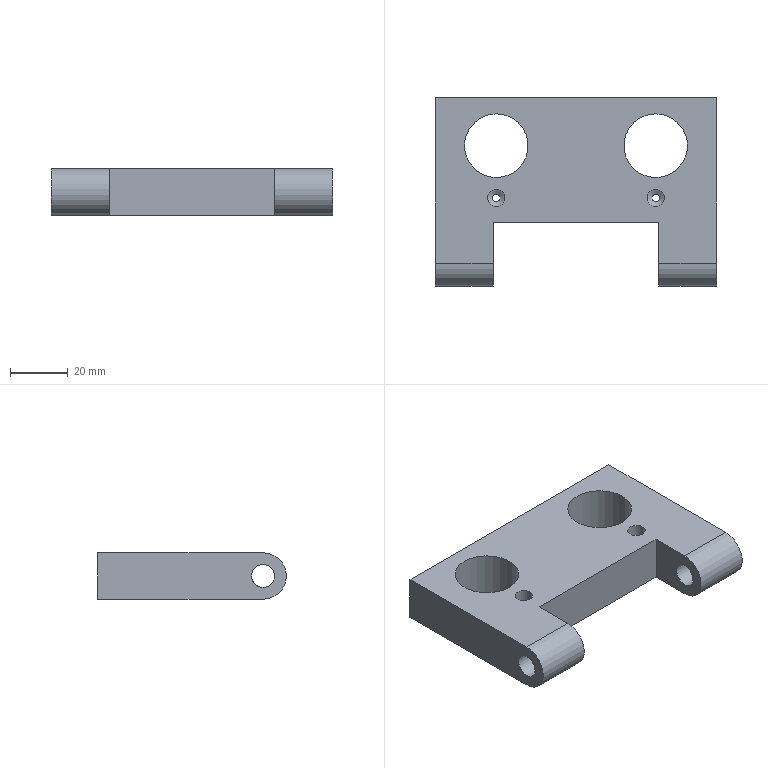Component | NX | DRILL_TEMPLATE | 1 solid | 18 faces | volume 64663 mm3 | plane 8 | cylinder 8 | cone 2 | commonest cylinder face diameters 16 x2 22 x2 8 x2 6 x2